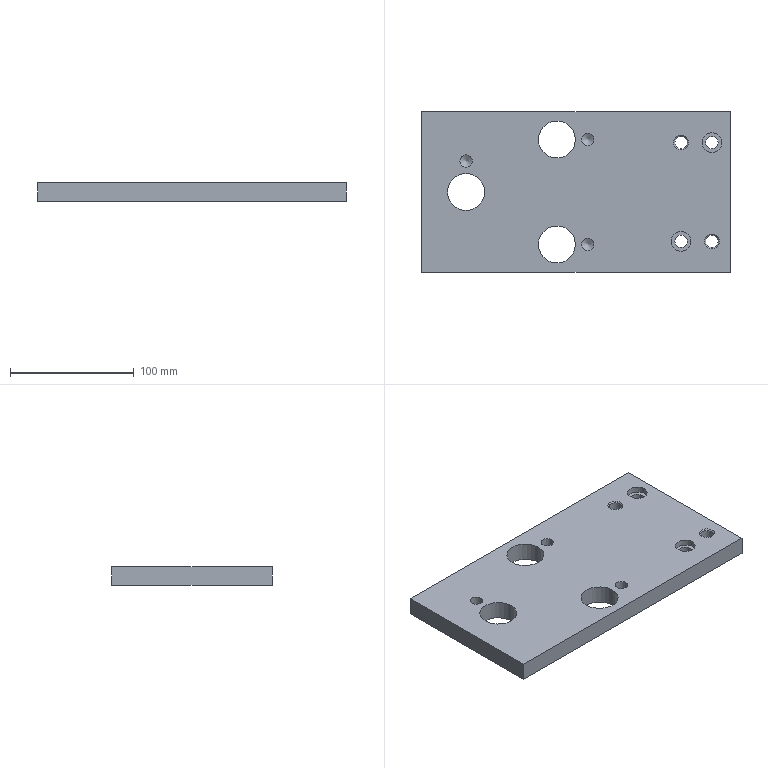Component | NX | GUIDE_PLATE | 1 solid | 25 faces | volume 447231 mm3 | cylinder 12 | plane 8 | cone 5 | commonest cylinder face diameters 10 x5 30 x3 16 x2 10.006 x2